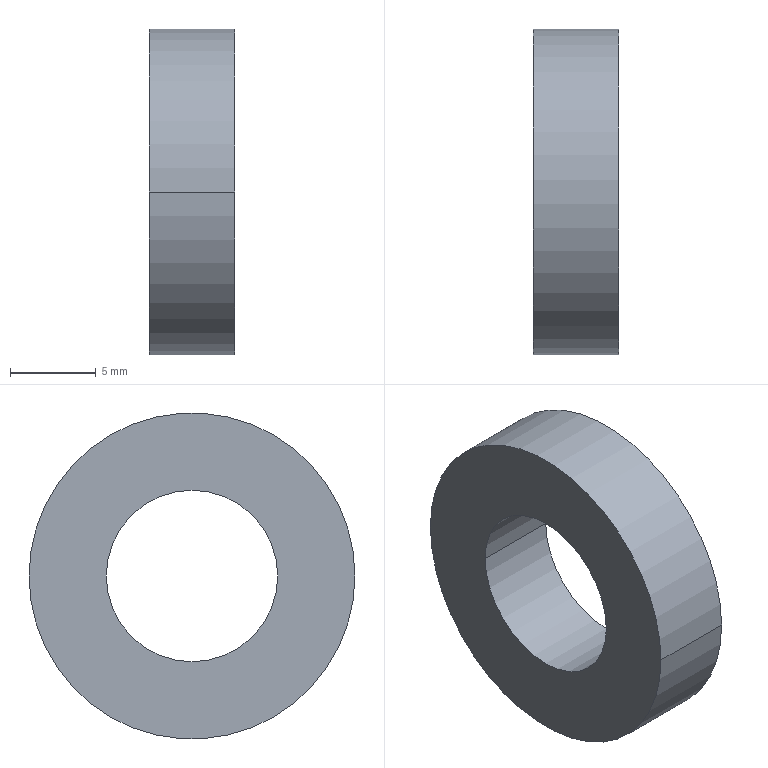Component | SolidWorks | 6800Bearing10-19-5-10 | 1 solid | 6 faces | box 5 x 19 x 19 mm | volume 1025 mm3 | cylinder 4 | plane 2 | commonest cylinder face diameters 10 x2 19 x2
build123d program:
from build123d import *

# Parameters (mm, degrees)
SKETCH1_R           = 9.5
SKETCH1_R_2         = 5
BOSS_EXTRUDE1_DEPTH = 2.5


with BuildPart() as part:
    # Sketch1 → Boss-Extrude1 (new, symmetric)
    with BuildSketch(Plane(origin=(0, 0, 0), x_dir=(0, 0, -1), z_dir=(1, 0, 0))):
        Circle(SKETCH1_R)
        Circle(SKETCH1_R_2, mode=Mode.SUBTRACT)
    extrude(amount=BOSS_EXTRUDE1_DEPTH, both=True)


solid = part.part

# Placed as in the assembly
solid = solid.moved(Location((204.5, 127.823, 79.212), (0, 0, 0)))
STEP:
#1=CARTESIAN_POINT('',(8.15,5.229,3.119));
#2=VERTEX_POINT('',#1);
#3=CARTESIAN_POINT('',(8.15,4.836,3.119));
#4=VERTEX_POINT('',#3);
#5=CARTESIAN_POINT('',(8.15,5.032,3.119));
#6=DIRECTION('',(1.,0.,-0.));
#7=DIRECTION('',(0.,-1.,0.));
#8=AXIS2_PLACEMENT_3D('',#5,#6,#7);
#9=CIRCLE('',#8,0.1969);
#10=EDGE_CURVE('',#2,#4,#9,.T.);
#11=ORIENTED_EDGE('',*,*,#10,.T.);
#12=CARTESIAN_POINT('',(7.953,4.836,3.119));
#13=VERTEX_POINT('',#12);
#14=CARTESIAN_POINT('',(8.15,4.836,3.119));
#15=DIRECTION('',(-1.,-0.,0.));
#16=VECTOR('',#15,39.37);
#17=LINE('',#14,#16);
#18=EDGE_CURVE('',#4,#13,#17,.T.);
#19=ORIENTED_EDGE('',*,*,#18,.T.);
#20=CARTESIAN_POINT('',(7.953,5.229,3.119));
#21=VERTEX_POINT('',#20);
#22=CARTESIAN_POINT('',(7.953,5.032,3.119));
#23=DIRECTION('',(1.,0.,-0.));
#24=DIRECTION('',(0.,-1.,0.));
#25=AXIS2_PLACEMENT_3D('',#22,#23,#24);
#26=CIRCLE('',#25,0.1969);
#27=EDGE_CURVE('',#21,#13,#26,.T.);
#28=ORIENTED_EDGE('',*,*,#27,.F.);
#29=CARTESIAN_POINT('',(8.15,5.229,3.119));
#30=DIRECTION('',(-1.,-0.,0.));
#31=VECTOR('',#30,39.37);
#32=LINE('',#29,#31);
#33=EDGE_CURVE('',#2,#21,#32,.T.);
#34=ORIENTED_EDGE('',*,*,#33,.F.);
#35=EDGE_LOOP('',(#11,#19,#28,#34));
#36=FACE_OUTER_BOUND('',#35,.T.);
#37=CARTESIAN_POINT('',(8.15,5.032,3.119));
#38=DIRECTION('',(-1.,-0.,0.));
#39=DIRECTION('',(0.,1.,0.));
#40=AXIS2_PLACEMENT_3D('',#37,#38,#39);
#41=CYLINDRICAL_SURFACE('',#40,0.1969);
#42=ADVANCED_FACE('',(#36),#41,.F.);
#43=CARTESIAN_POINT('',(8.15,4.658,3.119));
#44=VERTEX_POINT('',#43);
#45=CARTESIAN_POINT('',(8.15,5.406,3.119));
#46=VERTEX_POINT('',#45);
#47=CARTESIAN_POINT('',(8.15,5.032,3.119));
#48=DIRECTION('',(1.,0.,-0.));
#49=DIRECTION('',(0.,-1.,0.));
#50=AXIS2_PLACEMENT_3D('',#47,#48,#49);
#51=CIRCLE('',#50,0.374);
#52=EDGE_CURVE('',#44,#46,#51,.T.);
#53=ORIENTED_EDGE('',*,*,#52,.F.);
#54=CARTESIAN_POINT('',(7.953,4.658,3.119));
#55=VERTEX_POINT('',#54);
#56=CARTESIAN_POINT('',(8.15,4.658,3.119));
#57=DIRECTION('',(-1.,-0.,0.));
#58=VECTOR('',#57,39.37);
#59=LINE('',#56,#58);
#60=EDGE_CURVE('',#44,#55,#59,.T.);
#61=ORIENTED_EDGE('',*,*,#60,.T.);
#62=CARTESIAN_POINT('',(7.953,5.406,3.119));
#63=VERTEX_POINT('',#62);
#64=CARTESIAN_POINT('',(7.953,5.032,3.119));
#65=DIRECTION('',(1.,0.,-0.));
#66=DIRECTION('',(0.,-1.,0.));
#67=AXIS2_PLACEMENT_3D('',#64,#65,#66);
#68=CIRCLE('',#67,0.374);
#69=EDGE_CURVE('',#55,#63,#68,.T.);
#70=ORIENTED_EDGE('',*,*,#69,.T.);
#71=CARTESIAN_POINT('',(8.15,5.406,3.119));
#72=DIRECTION('',(-1.,-0.,0.));
#73=VECTOR('',#72,39.37);
#74=LINE('',#71,#73);
#75=EDGE_CURVE('',#46,#63,#74,.T.);
#76=ORIENTED_EDGE('',*,*,#75,.F.);
#77=EDGE_LOOP('',(#53,#61,#70,#76));
#78=FACE_OUTER_BOUND('',#77,.T.);
#79=CARTESIAN_POINT('',(8.15,5.032,3.119));
#80=DIRECTION('',(-1.,-0.,0.));
#81=DIRECTION('',(0.,1.,0.));
#82=AXIS2_PLACEMENT_3D('',#79,#80,#81);
#83=CYLINDRICAL_SURFACE('',#82,0.374);
#84=ADVANCED_FACE('',(#78),#83,.T.);
#85=CARTESIAN_POINT('',(8.15,5.032,3.119));
#86=DIRECTION('',(1.,0.,-0.));
#87=DIRECTION('',(0.,-1.,0.));
#88=AXIS2_PLACEMENT_3D('',#85,#86,#87);
#89=CIRCLE('',#88,0.374);
#90=EDGE_CURVE('',#46,#44,#89,.T.);
#91=ORIENTED_EDGE('',*,*,#90,.T.);
#92=ORIENTED_EDGE('',*,*,#52,.T.);
#93=EDGE_LOOP('',(#91,#92));
#94=FACE_OUTER_BOUND('',#93,.T.);
#95=ORIENTED_EDGE('',*,*,#10,.F.);
#96=CARTESIAN_POINT('',(8.15,5.032,3.119));
#97=DIRECTION('',(1.,0.,-0.));
#98=DIRECTION('',(0.,-1.,0.));
#99=AXIS2_PLACEMENT_3D('',#96,#97,#98);
#100=CIRCLE('',#99,0.1969);
#101=EDGE_CURVE('',#4,#2,#100,.T.);
#102=ORIENTED_EDGE('',*,*,#101,.F.);
#103=EDGE_LOOP('',(#95,#102));
#104=FACE_BOUND('',#103,.T.);
#105=CARTESIAN_POINT('',(8.15,5.032,3.119));
#106=DIRECTION('',(1.,0.,-0.));
#107=DIRECTION('',(0.,-1.,-0.));
#108=AXIS2_PLACEMENT_3D('',#105,#106,#107);
#109=PLANE('',#108);
#110=ADVANCED_FACE('',(#94,#104),#109,.T.);
#111=CARTESIAN_POINT('',(7.953,5.032,3.119));
#112=DIRECTION('',(1.,0.,-0.));
#113=DIRECTION('',(0.,-1.,0.));
#114=AXIS2_PLACEMENT_3D('',#111,#112,#113);
#115=CIRCLE('',#114,0.374);
#116=EDGE_CURVE('',#63,#55,#115,.T.);
#117=ORIENTED_EDGE('',*,*,#116,.F.);
#118=ORIENTED_EDGE('',*,*,#69,.F.);
#119=EDGE_LOOP('',(#117,#118));
#120=FACE_OUTER_BOUND('',#119,.T.);
#121=ORIENTED_EDGE('',*,*,#27,.T.);
#122=CARTESIAN_POINT('',(7.953,5.032,3.119));
#123=DIRECTION('',(1.,0.,-0.));
#124=DIRECTION('',(0.,-1.,0.));
#125=AXIS2_PLACEMENT_3D('',#122,#123,#124);
#126=CIRCLE('',#125,0.1969);
#127=EDGE_CURVE('',#13,#21,#126,.T.);
#128=ORIENTED_EDGE('',*,*,#127,.T.);
#129=EDGE_LOOP('',(#121,#128));
#130=FACE_BOUND('',#129,.T.);
#131=CARTESIAN_POINT('',(7.953,5.032,3.119));
#132=DIRECTION('',(1.,0.,-0.));
#133=DIRECTION('',(0.,-1.,-0.));
#134=AXIS2_PLACEMENT_3D('',#131,#132,#133);
#135=PLANE('',#134);
#136=ADVANCED_FACE('',(#120,#130),#135,.F.);
#137=ORIENTED_EDGE('',*,*,#60,.F.);
#138=ORIENTED_EDGE('',*,*,#90,.F.);
#139=ORIENTED_EDGE('',*,*,#75,.T.);
#140=ORIENTED_EDGE('',*,*,#116,.T.);
#141=EDGE_LOOP('',(#137,#138,#139,#140));
#142=FACE_OUTER_BOUND('',#141,.T.);
#143=CARTESIAN_POINT('',(8.15,5.032,3.119));
#144=DIRECTION('',(-1.,-0.,0.));
#145=DIRECTION('',(0.,1.,0.));
#146=AXIS2_PLACEMENT_3D('',#143,#144,#145);
#147=CYLINDRICAL_SURFACE('',#146,0.374);
#148=ADVANCED_FACE('',(#142),#147,.T.);
#149=ORIENTED_EDGE('',*,*,#18,.F.);
#150=ORIENTED_EDGE('',*,*,#101,.T.);
#151=ORIENTED_EDGE('',*,*,#33,.T.);
#152=ORIENTED_EDGE('',*,*,#127,.F.);
#153=EDGE_LOOP('',(#149,#150,#151,#152));
#154=FACE_OUTER_BOUND('',#153,.T.);
#155=CARTESIAN_POINT('',(8.15,5.032,3.119));
#156=DIRECTION('',(-1.,-0.,0.));
#157=DIRECTION('',(0.,1.,0.));
#158=AXIS2_PLACEMENT_3D('',#155,#156,#157);
#159=CYLINDRICAL_SURFACE('',#158,0.1969);
#160=ADVANCED_FACE('',(#154),#159,.F.);
#161=CLOSED_SHELL('',(#42,#84,#110,#136,#148,#160));
#162=MANIFOLD_SOLID_BREP('',#161);
#163=CARTESIAN_POINT('',(0.,0.,0.));
#164=DIRECTION('',(0.,0.,1.));
#165=DIRECTION('',(1.,0.,0.));
#166=AXIS2_PLACEMENT_3D('',#163,#164,#165);
#167=(LENGTH_UNIT()NAMED_UNIT(*)SI_UNIT($,.METRE.));
#168=LENGTH_MEASURE_WITH_UNIT(LENGTH_MEASURE(0.0254),#167);
#169=DIMENSIONAL_EXPONENTS(1.,0.,0.,0.,0.,0.,0.);
#170=(CONVERSION_BASED_UNIT('',#168)LENGTH_UNIT()NAMED_UNIT(#169));
#171=UNCERTAINTY_MEASURE_WITH_UNIT(LENGTH_MEASURE(0.00001),#170,'','');
#172=(NAMED_UNIT(*)PLANE_ANGLE_UNIT()SI_UNIT($,.RADIAN.));
#173=(NAMED_UNIT(*)SI_UNIT($,.STERADIAN.)SOLID_ANGLE_UNIT());
#174=(GEOMETRIC_REPRESENTATION_CONTEXT(3)GLOBAL_UNCERTAINTY_ASSIGNED_CONTEXT((#171))GLOBAL_UNIT_ASSIGNED_CONTEXT((#170,#172,#173))REPRESENTATION_CONTEXT('',''));
#175=ADVANCED_BREP_SHAPE_REPRESENTATION('',(#162,#166),#174);
#176=COLOUR_RGB('',0.7922,0.8196,0.9333);
#177=FILL_AREA_STYLE_COLOUR('',#176);
#178=FILL_AREA_STYLE('',(#177));
#179=SURFACE_STYLE_FILL_AREA(#178);
#180=SURFACE_SIDE_STYLE('',(#179));
#181=SURFACE_STYLE_USAGE(.BOTH.,#180);
#182=PRESENTATION_STYLE_ASSIGNMENT((#181));
#183=STYLED_ITEM('',(#182),#162);
#184=(LENGTH_UNIT()NAMED_UNIT(*)SI_UNIT($,.METRE.));
#185=LENGTH_MEASURE_WITH_UNIT(LENGTH_MEASURE(0.0254),#184);
#186=DIMENSIONAL_EXPONENTS(1.,0.,0.,0.,0.,0.,0.);
#187=(CONVERSION_BASED_UNIT('',#185)LENGTH_UNIT()NAMED_UNIT(#186));
#188=UNCERTAINTY_MEASURE_WITH_UNIT(LENGTH_MEASURE(0.00001),#187,'','');
#189=(NAMED_UNIT(*)PLANE_ANGLE_UNIT()SI_UNIT($,.RADIAN.));
#190=(NAMED_UNIT(*)SI_UNIT($,.STERADIAN.)SOLID_ANGLE_UNIT());
#191=(GEOMETRIC_REPRESENTATION_CONTEXT(3)GLOBAL_UNCERTAINTY_ASSIGNED_CONTEXT((#188))GLOBAL_UNIT_ASSIGNED_CONTEXT((#187,#189,#190))REPRESENTATION_CONTEXT('',''));
#192=MECHANICAL_DESIGN_GEOMETRIC_PRESENTATION_REPRESENTATION('',(#183),#191);
#193=PRESENTATION_LAYER_ASSIGNMENT('','',(#183));